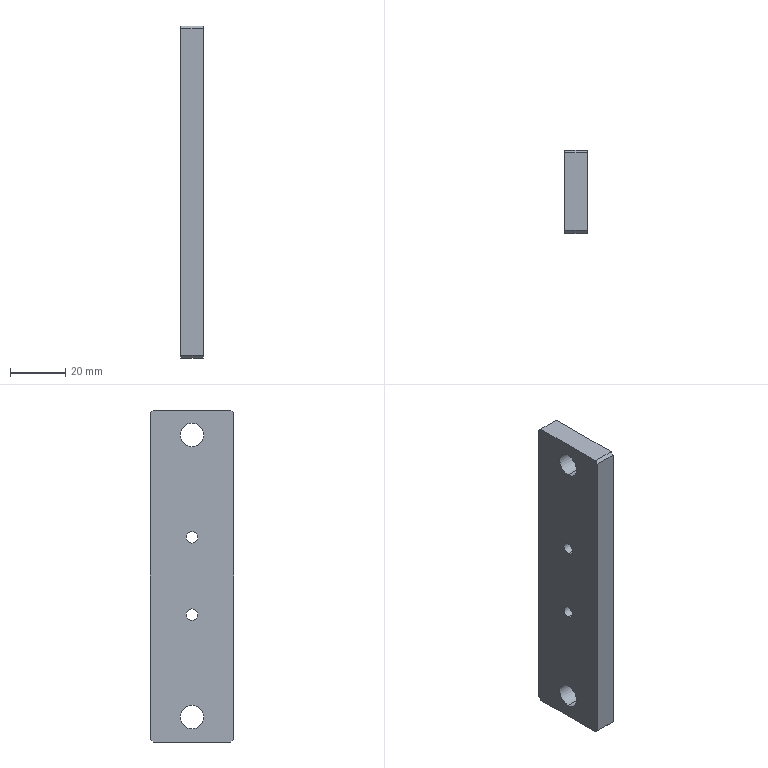Component | SolidWorks | LH-CGJ-01-055-1 | 1 solid | 18 faces | box 8 x 30 x 120 mm | volume 27654 mm3 | plane 10 | cylinder 8 | commonest cylinder face diameters 8.5 x4 4.2 x4 | material A6061
build123d program:
from build123d import *

# Parameters (mm, degrees)
SKETCH1_W                      = 120
SKETCH1_H                      = 30
BOSS_EXTRUDE1_DEPTH            = 8
M5_TAPPED_HOLE1_D              = 4.2
M5_TAPPED_HOLE1_DEPTH          = 12.4
M5_TAPPED_HOLE1_TIP            = 1.262
CHAMFER1_SIZE                  = 1
F_8_5_8_5_DIAMETER_HOLE1_D     = 8.5
F_8_5_8_5_DIAMETER_HOLE1_DEPTH = 12.4
F_8_5_8_5_DIAMETER_HOLE1_TIP   = 2.554


with BuildPart() as part:
    # Sketch1 → Boss-Extrude1 (new body)
    with BuildSketch(Plane.XY):
        with Locations((60, 15)):
            Rectangle(SKETCH1_W, SKETCH1_H)
    extrude(amount=BOSS_EXTRUDE1_DEPTH)

    # M5 Tapped Hole1
    with Locations(Plane.XY.offset(8)):
        with Locations((46, 15), (74, 15)):
            Hole(M5_TAPPED_HOLE1_D / 2, depth=M5_TAPPED_HOLE1_DEPTH)
            with Locations((0, 0, -(M5_TAPPED_HOLE1_DEPTH + M5_TAPPED_HOLE1_TIP / 2))):  # 118° drill point
                Cone(0, M5_TAPPED_HOLE1_D / 2, M5_TAPPED_HOLE1_TIP, mode=Mode.SUBTRACT)

    # Chamfer1
    chamfer1_edges = [part.edges().sort_by_distance(p)[0] for p in [
        (0, 30, 4),
        (120, 30, 4),
        (120, 0, 4),
        (0, 0, 4),
    ]]
    chamfer(chamfer1_edges, length=CHAMFER1_SIZE)

    # 8.5 _8.5_ Diameter Hole1
    with Locations(Plane(origin=(0, 0, 0), x_dir=(-1, 0, 0), z_dir=(0, 0, -1))):
        with Locations((-9, 15), (-111, 15)):
            Hole(F_8_5_8_5_DIAMETER_HOLE1_D / 2, depth=F_8_5_8_5_DIAMETER_HOLE1_DEPTH)
            with Locations((0, 0, -(F_8_5_8_5_DIAMETER_HOLE1_DEPTH + F_8_5_8_5_DIAMETER_HOLE1_TIP / 2))):  # 118° drill point
                Cone(0, F_8_5_8_5_DIAMETER_HOLE1_D / 2, F_8_5_8_5_DIAMETER_HOLE1_TIP, mode=Mode.SUBTRACT)


solid = part.part

# Placed as in the assembly
solid = solid.moved(Location((-38.503, 90.215, 125.05), (0, 90, 0)))
STEP:
#1=COLOUR_RGB('',0.7922,0.8196,0.9333);
#2=FILL_AREA_STYLE_COLOUR('',#1);
#3=FILL_AREA_STYLE('',(#2));
#4=SURFACE_STYLE_FILL_AREA(#3);
#5=SURFACE_SIDE_STYLE('',(#4));
#6=SURFACE_STYLE_USAGE(.BOTH.,#5);
#7=PRESENTATION_STYLE_ASSIGNMENT((#6));
#8=CARTESIAN_POINT('',(-1.516,4.142,0.7205));
#9=VERTEX_POINT('',#8);
#10=CARTESIAN_POINT('',(-1.516,4.142,0.3858));
#11=VERTEX_POINT('',#10);
#12=CARTESIAN_POINT('',(-1.516,4.142,0.5531));
#13=DIRECTION('',(1.,0.,-0.));
#14=DIRECTION('',(0.,0.,-1.));
#15=AXIS2_PLACEMENT_3D('',#12,#13,#14);
#16=CIRCLE('',#15,0.1673);
#17=EDGE_CURVE('',#9,#11,#16,.T.);
#18=ORIENTED_EDGE('',*,*,#17,.F.);
#19=CARTESIAN_POINT('',(-1.201,4.142,0.7205));
#20=VERTEX_POINT('',#19);
#21=CARTESIAN_POINT('',(-1.201,4.142,0.7205));
#22=DIRECTION('',(1.,0.,-0.));
#23=VECTOR('',#22,39.37);
#24=LINE('',#21,#23);
#25=EDGE_CURVE('',#9,#20,#24,.T.);
#26=ORIENTED_EDGE('',*,*,#25,.T.);
#27=CARTESIAN_POINT('',(-1.201,4.142,0.3858));
#28=VERTEX_POINT('',#27);
#29=CARTESIAN_POINT('',(-1.201,4.142,0.5531));
#30=DIRECTION('',(1.,0.,-0.));
#31=DIRECTION('',(-0.,0.,-1.));
#32=AXIS2_PLACEMENT_3D('',#29,#30,#31);
#33=CIRCLE('',#32,0.1673);
#34=EDGE_CURVE('',#20,#28,#33,.T.);
#35=ORIENTED_EDGE('',*,*,#34,.T.);
#36=CARTESIAN_POINT('',(-1.201,4.142,0.3858));
#37=DIRECTION('',(1.,0.,-0.));
#38=VECTOR('',#37,39.37);
#39=LINE('',#36,#38);
#40=EDGE_CURVE('',#11,#28,#39,.T.);
#41=ORIENTED_EDGE('',*,*,#40,.F.);
#42=EDGE_LOOP('',(#18,#26,#35,#41));
#43=FACE_OUTER_BOUND('',#42,.T.);
#44=CARTESIAN_POINT('',(-1.201,4.142,0.5531));
#45=DIRECTION('',(1.,0.,-0.));
#46=DIRECTION('',(-0.,0.,-1.));
#47=AXIS2_PLACEMENT_3D('',#44,#45,#46);
#48=CYLINDRICAL_SURFACE('',#47,0.1673);
#49=ADVANCED_FACE('',(#43),#48,.F.);
#50=CARTESIAN_POINT('',(-1.516,4.142,4.736));
#51=VERTEX_POINT('',#50);
#52=CARTESIAN_POINT('',(-1.516,4.142,4.402));
#53=VERTEX_POINT('',#52);
#54=CARTESIAN_POINT('',(-1.516,4.142,4.569));
#55=DIRECTION('',(1.,0.,-0.));
#56=DIRECTION('',(0.,0.,-1.));
#57=AXIS2_PLACEMENT_3D('',#54,#55,#56);
#58=CIRCLE('',#57,0.1673);
#59=EDGE_CURVE('',#51,#53,#58,.T.);
#60=ORIENTED_EDGE('',*,*,#59,.F.);
#61=CARTESIAN_POINT('',(-1.201,4.142,4.736));
#62=VERTEX_POINT('',#61);
#63=CARTESIAN_POINT('',(-1.201,4.142,4.736));
#64=DIRECTION('',(1.,0.,-0.));
#65=VECTOR('',#64,39.37);
#66=LINE('',#63,#65);
#67=EDGE_CURVE('',#51,#62,#66,.T.);
#68=ORIENTED_EDGE('',*,*,#67,.T.);
#69=CARTESIAN_POINT('',(-1.201,4.142,4.402));
#70=VERTEX_POINT('',#69);
#71=CARTESIAN_POINT('',(-1.201,4.142,4.569));
#72=DIRECTION('',(1.,0.,-0.));
#73=DIRECTION('',(-0.,0.,-1.));
#74=AXIS2_PLACEMENT_3D('',#71,#72,#73);
#75=CIRCLE('',#74,0.1673);
#76=EDGE_CURVE('',#62,#70,#75,.T.);
#77=ORIENTED_EDGE('',*,*,#76,.T.);
#78=CARTESIAN_POINT('',(-1.201,4.142,4.402));
#79=DIRECTION('',(1.,0.,-0.));
#80=VECTOR('',#79,39.37);
#81=LINE('',#78,#80);
#82=EDGE_CURVE('',#53,#70,#81,.T.);
#83=ORIENTED_EDGE('',*,*,#82,.F.);
#84=EDGE_LOOP('',(#60,#68,#77,#83));
#85=FACE_OUTER_BOUND('',#84,.T.);
#86=CARTESIAN_POINT('',(-1.201,4.142,4.569));
#87=DIRECTION('',(1.,0.,-0.));
#88=DIRECTION('',(-0.,0.,-1.));
#89=AXIS2_PLACEMENT_3D('',#86,#87,#88);
#90=CYLINDRICAL_SURFACE('',#89,0.1673);
#91=ADVANCED_FACE('',(#85),#90,.F.);
#92=CARTESIAN_POINT('',(-1.201,4.142,2.093));
#93=VERTEX_POINT('',#92);
#94=CARTESIAN_POINT('',(-1.201,4.142,1.927));
#95=VERTEX_POINT('',#94);
#96=CARTESIAN_POINT('',(-1.201,4.142,2.01));
#97=DIRECTION('',(1.,0.,-0.));
#98=DIRECTION('',(0.,0.,-1.));
#99=AXIS2_PLACEMENT_3D('',#96,#97,#98);
#100=CIRCLE('',#99,0.08268);
#101=EDGE_CURVE('',#93,#95,#100,.T.);
#102=ORIENTED_EDGE('',*,*,#101,.T.);
#103=CARTESIAN_POINT('',(-1.516,4.142,1.927));
#104=VERTEX_POINT('',#103);
#105=CARTESIAN_POINT('',(-1.516,4.142,1.927));
#106=DIRECTION('',(-1.,-0.,0.));
#107=VECTOR('',#106,39.37);
#108=LINE('',#105,#107);
#109=EDGE_CURVE('',#95,#104,#108,.T.);
#110=ORIENTED_EDGE('',*,*,#109,.T.);
#111=CARTESIAN_POINT('',(-1.516,4.142,2.093));
#112=VERTEX_POINT('',#111);
#113=CARTESIAN_POINT('',(-1.516,4.142,2.01));
#114=DIRECTION('',(-1.,-0.,0.));
#115=DIRECTION('',(0.,0.,1.));
#116=AXIS2_PLACEMENT_3D('',#113,#114,#115);
#117=CIRCLE('',#116,0.08268);
#118=EDGE_CURVE('',#104,#112,#117,.T.);
#119=ORIENTED_EDGE('',*,*,#118,.T.);
#120=CARTESIAN_POINT('',(-1.516,4.142,2.093));
#121=DIRECTION('',(-1.,-0.,0.));
#122=VECTOR('',#121,39.37);
#123=LINE('',#120,#122);
#124=EDGE_CURVE('',#93,#112,#123,.T.);
#125=ORIENTED_EDGE('',*,*,#124,.F.);
#126=EDGE_LOOP('',(#102,#110,#119,#125));
#127=FACE_OUTER_BOUND('',#126,.T.);
#128=CARTESIAN_POINT('',(-1.516,4.142,2.01));
#129=DIRECTION('',(-1.,-0.,0.));
#130=DIRECTION('',(0.,0.,1.));
#131=AXIS2_PLACEMENT_3D('',#128,#129,#130);
#132=CYLINDRICAL_SURFACE('',#131,0.08268);
#133=ADVANCED_FACE('',(#127),#132,.F.);
#134=CARTESIAN_POINT('',(-1.201,4.142,3.195));
#135=VERTEX_POINT('',#134);
#136=CARTESIAN_POINT('',(-1.201,4.142,3.03));
#137=VERTEX_POINT('',#136);
#138=CARTESIAN_POINT('',(-1.201,4.142,3.112));
#139=DIRECTION('',(1.,0.,-0.));
#140=DIRECTION('',(0.,0.,-1.));
#141=AXIS2_PLACEMENT_3D('',#138,#139,#140);
#142=CIRCLE('',#141,0.08268);
#143=EDGE_CURVE('',#135,#137,#142,.T.);
#144=ORIENTED_EDGE('',*,*,#143,.T.);
#145=CARTESIAN_POINT('',(-1.516,4.142,3.03));
#146=VERTEX_POINT('',#145);
#147=CARTESIAN_POINT('',(-1.516,4.142,3.03));
#148=DIRECTION('',(-1.,-0.,0.));
#149=VECTOR('',#148,39.37);
#150=LINE('',#147,#149);
#151=EDGE_CURVE('',#137,#146,#150,.T.);
#152=ORIENTED_EDGE('',*,*,#151,.T.);
#153=CARTESIAN_POINT('',(-1.516,4.142,3.195));
#154=VERTEX_POINT('',#153);
#155=CARTESIAN_POINT('',(-1.516,4.142,3.112));
#156=DIRECTION('',(-1.,-0.,0.));
#157=DIRECTION('',(0.,0.,1.));
#158=AXIS2_PLACEMENT_3D('',#155,#156,#157);
#159=CIRCLE('',#158,0.08268);
#160=EDGE_CURVE('',#146,#154,#159,.T.);
#161=ORIENTED_EDGE('',*,*,#160,.T.);
#162=CARTESIAN_POINT('',(-1.516,4.142,3.195));
#163=DIRECTION('',(-1.,-0.,0.));
#164=VECTOR('',#163,39.37);
#165=LINE('',#162,#164);
#166=EDGE_CURVE('',#135,#154,#165,.T.);
#167=ORIENTED_EDGE('',*,*,#166,.F.);
#168=EDGE_LOOP('',(#144,#152,#161,#167));
#169=FACE_OUTER_BOUND('',#168,.T.);
#170=CARTESIAN_POINT('',(-1.516,4.142,3.112));
#171=DIRECTION('',(-1.,-0.,0.));
#172=DIRECTION('',(0.,0.,1.));
#173=AXIS2_PLACEMENT_3D('',#170,#171,#172);
#174=CYLINDRICAL_SURFACE('',#173,0.08268);
#175=ADVANCED_FACE('',(#169),#174,.F.);
#176=CARTESIAN_POINT('',(-1.201,4.694,0.1988));
#177=VERTEX_POINT('',#176);
#178=CARTESIAN_POINT('',(-1.201,3.591,0.1988));
#179=VERTEX_POINT('',#178);
#180=CARTESIAN_POINT('',(-1.201,3.552,0.1988));
#181=DIRECTION('',(0.,-1.,-0.));
#182=VECTOR('',#181,39.37);
#183=LINE('',#180,#182);
#184=EDGE_CURVE('',#177,#179,#183,.T.);
#185=ORIENTED_EDGE('',*,*,#184,.T.);
#186=CARTESIAN_POINT('',(-1.516,3.591,0.1988));
#187=VERTEX_POINT('',#186);
#188=CARTESIAN_POINT('',(-1.516,3.591,0.1988));
#189=DIRECTION('',(-1.,-0.,0.));
#190=VECTOR('',#189,39.37);
#191=LINE('',#188,#190);
#192=EDGE_CURVE('',#179,#187,#191,.T.);
#193=ORIENTED_EDGE('',*,*,#192,.T.);
#194=CARTESIAN_POINT('',(-1.516,4.694,0.1988));
#195=VERTEX_POINT('',#194);
#196=CARTESIAN_POINT('',(-1.516,3.552,0.1988));
#197=DIRECTION('',(0.,-1.,-0.));
#198=VECTOR('',#197,39.37);
#199=LINE('',#196,#198);
#200=EDGE_CURVE('',#195,#187,#199,.T.);
#201=ORIENTED_EDGE('',*,*,#200,.F.);
#202=CARTESIAN_POINT('',(-1.516,4.694,0.1988));
#203=DIRECTION('',(1.,0.,-0.));
#204=VECTOR('',#203,39.37);
#205=LINE('',#202,#204);
#206=EDGE_CURVE('',#195,#177,#205,.T.);
#207=ORIENTED_EDGE('',*,*,#206,.T.);
#208=EDGE_LOOP('',(#185,#193,#201,#207));
#209=FACE_OUTER_BOUND('',#208,.T.);
#210=CARTESIAN_POINT('',(-1.516,3.552,0.1988));
#211=DIRECTION('',(0.,-0.,1.));
#212=DIRECTION('',(1.,0.,-0.));
#213=AXIS2_PLACEMENT_3D('',#210,#211,#212);
#214=PLANE('',#213);
#215=ADVANCED_FACE('',(#209),#214,.F.);
#216=CARTESIAN_POINT('',(-1.516,3.552,0.2382));
#217=VERTEX_POINT('',#216);
#218=CARTESIAN_POINT('',(-1.516,3.552,4.884));
#219=VERTEX_POINT('',#218);
#220=CARTESIAN_POINT('',(-1.516,3.552,0.1988));
#221=DIRECTION('',(0.,-0.,1.));
#222=VECTOR('',#221,39.37);
#223=LINE('',#220,#222);
#224=EDGE_CURVE('',#217,#219,#223,.T.);
#225=ORIENTED_EDGE('',*,*,#224,.F.);
#226=CARTESIAN_POINT('',(-1.201,3.552,0.2382));
#227=VERTEX_POINT('',#226);
#228=CARTESIAN_POINT('',(-1.516,3.552,0.2382));
#229=DIRECTION('',(1.,0.,-0.));
#230=VECTOR('',#229,39.37);
#231=LINE('',#228,#230);
#232=EDGE_CURVE('',#217,#227,#231,.T.);
#233=ORIENTED_EDGE('',*,*,#232,.T.);
#234=CARTESIAN_POINT('',(-1.201,3.552,4.884));
#235=VERTEX_POINT('',#234);
#236=CARTESIAN_POINT('',(-1.201,3.552,0.1988));
#237=DIRECTION('',(0.,-0.,1.));
#238=VECTOR('',#237,39.37);
#239=LINE('',#236,#238);
#240=EDGE_CURVE('',#227,#235,#239,.T.);
#241=ORIENTED_EDGE('',*,*,#240,.T.);
#242=CARTESIAN_POINT('',(-1.516,3.552,4.884));
#243=DIRECTION('',(-1.,-0.,0.));
#244=VECTOR('',#243,39.37);
#245=LINE('',#242,#244);
#246=EDGE_CURVE('',#235,#219,#245,.T.);
#247=ORIENTED_EDGE('',*,*,#246,.T.);
#248=EDGE_LOOP('',(#225,#233,#241,#247));
#249=FACE_OUTER_BOUND('',#248,.T.);
#250=CARTESIAN_POINT('',(-1.516,3.552,0.1988));
#251=DIRECTION('',(-0.,1.,0.));
#252=DIRECTION('',(-1.,-0.,0.));
#253=AXIS2_PLACEMENT_3D('',#250,#251,#252);
#254=PLANE('',#253);
#255=ADVANCED_FACE('',(#249),#254,.F.);
#256=CARTESIAN_POINT('',(-1.516,3.591,4.923));
#257=VERTEX_POINT('',#256);
#258=CARTESIAN_POINT('',(-1.516,4.694,4.923));
#259=VERTEX_POINT('',#258);
#260=CARTESIAN_POINT('',(-1.516,3.552,4.923));
#261=DIRECTION('',(-0.,1.,0.));
#262=VECTOR('',#261,39.37);
#263=LINE('',#260,#262);
#264=EDGE_CURVE('',#257,#259,#263,.T.);
#265=ORIENTED_EDGE('',*,*,#264,.F.);
#266=CARTESIAN_POINT('',(-1.201,3.591,4.923));
#267=VERTEX_POINT('',#266);
#268=CARTESIAN_POINT('',(-1.516,3.591,4.923));
#269=DIRECTION('',(1.,0.,-0.));
#270=VECTOR('',#269,39.37);
#271=LINE('',#268,#270);
#272=EDGE_CURVE('',#257,#267,#271,.T.);
#273=ORIENTED_EDGE('',*,*,#272,.T.);
#274=CARTESIAN_POINT('',(-1.201,4.694,4.923));
#275=VERTEX_POINT('',#274);
#276=CARTESIAN_POINT('',(-1.201,3.552,4.923));
#277=DIRECTION('',(-0.,1.,0.));
#278=VECTOR('',#277,39.37);
#279=LINE('',#276,#278);
#280=EDGE_CURVE('',#267,#275,#279,.T.);
#281=ORIENTED_EDGE('',*,*,#280,.T.);
#282=CARTESIAN_POINT('',(-1.516,4.694,4.923));
#283=DIRECTION('',(-1.,-0.,0.));
#284=VECTOR('',#283,39.37);
#285=LINE('',#282,#284);
#286=EDGE_CURVE('',#275,#259,#285,.T.);
#287=ORIENTED_EDGE('',*,*,#286,.T.);
#288=EDGE_LOOP('',(#265,#273,#281,#287));
#289=FACE_OUTER_BOUND('',#288,.T.);
#290=CARTESIAN_POINT('',(-1.516,3.552,4.923));
#291=DIRECTION('',(-0.,0.,-1.));
#292=DIRECTION('',(-1.,-0.,0.));
#293=AXIS2_PLACEMENT_3D('',#290,#291,#292);
#294=PLANE('',#293);
#295=ADVANCED_FACE('',(#289),#294,.F.);
#296=CARTESIAN_POINT('',(-1.201,4.733,4.884));
#297=VERTEX_POINT('',#296);
#298=CARTESIAN_POINT('',(-1.201,4.733,0.2382));
#299=VERTEX_POINT('',#298);
#300=CARTESIAN_POINT('',(-1.201,4.733,0.1988));
#301=DIRECTION('',(-0.,0.,-1.));
#302=VECTOR('',#301,39.37);
#303=LINE('',#300,#302);
#304=EDGE_CURVE('',#297,#299,#303,.T.);
#305=ORIENTED_EDGE('',*,*,#304,.T.);
#306=CARTESIAN_POINT('',(-1.516,4.733,0.2382));
#307=VERTEX_POINT('',#306);
#308=CARTESIAN_POINT('',(-1.516,4.733,0.2382));
#309=DIRECTION('',(-1.,-0.,0.));
#310=VECTOR('',#309,39.37);
#311=LINE('',#308,#310);
#312=EDGE_CURVE('',#299,#307,#311,.T.);
#313=ORIENTED_EDGE('',*,*,#312,.T.);
#314=CARTESIAN_POINT('',(-1.516,4.733,4.884));
#315=VERTEX_POINT('',#314);
#316=CARTESIAN_POINT('',(-1.516,4.733,0.1988));
#317=DIRECTION('',(-0.,0.,-1.));
#318=VECTOR('',#317,39.37);
#319=LINE('',#316,#318);
#320=EDGE_CURVE('',#315,#307,#319,.T.);
#321=ORIENTED_EDGE('',*,*,#320,.F.);
#322=CARTESIAN_POINT('',(-1.516,4.733,4.884));
#323=DIRECTION('',(1.,0.,-0.));
#324=VECTOR('',#323,39.37);
#325=LINE('',#322,#324);
#326=EDGE_CURVE('',#315,#297,#325,.T.);
#327=ORIENTED_EDGE('',*,*,#326,.T.);
#328=EDGE_LOOP('',(#305,#313,#321,#327));
#329=FACE_OUTER_BOUND('',#328,.T.);
#330=CARTESIAN_POINT('',(-1.516,4.733,0.1988));
#331=DIRECTION('',(0.,-1.,-0.));
#332=DIRECTION('',(1.,0.,-0.));
#333=AXIS2_PLACEMENT_3D('',#330,#331,#332);
#334=PLANE('',#333);
#335=ADVANCED_FACE('',(#329),#334,.F.);
#336=CARTESIAN_POINT('',(-1.516,4.142,0.5531));
#337=DIRECTION('',(1.,0.,-0.));
#338=DIRECTION('',(0.,0.,-1.));
#339=AXIS2_PLACEMENT_3D('',#336,#337,#338);
#340=CIRCLE('',#339,0.1673);
#341=EDGE_CURVE('',#11,#9,#340,.T.);
#342=ORIENTED_EDGE('',*,*,#341,.T.);
#343=ORIENTED_EDGE('',*,*,#17,.T.);
#344=EDGE_LOOP('',(#342,#343));
#345=FACE_BOUND('',#344,.T.);
#346=CARTESIAN_POINT('',(-1.516,4.142,4.569));
#347=DIRECTION('',(1.,0.,-0.));
#348=DIRECTION('',(0.,0.,-1.));
#349=AXIS2_PLACEMENT_3D('',#346,#347,#348);
#350=CIRCLE('',#349,0.1673);
#351=EDGE_CURVE('',#53,#51,#350,.T.);
#352=ORIENTED_EDGE('',*,*,#351,.T.);
#353=ORIENTED_EDGE('',*,*,#59,.T.);
#354=EDGE_LOOP('',(#352,#353));
#355=FACE_BOUND('',#354,.T.);
#356=CARTESIAN_POINT('',(-1.516,4.142,2.01));
#357=DIRECTION('',(-1.,-0.,0.));
#358=DIRECTION('',(0.,0.,1.));
#359=AXIS2_PLACEMENT_3D('',#356,#357,#358);
#360=CIRCLE('',#359,0.08268);
#361=EDGE_CURVE('',#112,#104,#360,.T.);
#362=ORIENTED_EDGE('',*,*,#361,.F.);
#363=ORIENTED_EDGE('',*,*,#118,.F.);
#364=EDGE_LOOP('',(#362,#363));
#365=FACE_BOUND('',#364,.T.);
#366=CARTESIAN_POINT('',(-1.516,4.142,3.112));
#367=DIRECTION('',(-1.,-0.,0.));
#368=DIRECTION('',(0.,0.,1.));
#369=AXIS2_PLACEMENT_3D('',#366,#367,#368);
#370=CIRCLE('',#369,0.08268);
#371=EDGE_CURVE('',#154,#146,#370,.T.);
#372=ORIENTED_EDGE('',*,*,#371,.F.);
#373=ORIENTED_EDGE('',*,*,#160,.F.);
#374=EDGE_LOOP('',(#372,#373));
#375=FACE_BOUND('',#374,.T.);
#376=ORIENTED_EDGE('',*,*,#200,.T.);
#377=CARTESIAN_POINT('',(-1.516,3.552,0.2382));
#378=DIRECTION('',(0.,-0.7071,0.7071));
#379=VECTOR('',#378,39.37);
#380=LINE('',#377,#379);
#381=EDGE_CURVE('',#187,#217,#380,.T.);
#382=ORIENTED_EDGE('',*,*,#381,.T.);
#383=ORIENTED_EDGE('',*,*,#224,.T.);
#384=CARTESIAN_POINT('',(-1.516,3.591,4.923));
#385=DIRECTION('',(0.,0.7071,0.7071));
#386=VECTOR('',#385,39.37);
#387=LINE('',#384,#386);
#388=EDGE_CURVE('',#219,#257,#387,.T.);
#389=ORIENTED_EDGE('',*,*,#388,.T.);
#390=ORIENTED_EDGE('',*,*,#264,.T.);
#391=CARTESIAN_POINT('',(-1.516,4.733,4.884));
#392=DIRECTION('',(-0.,0.7071,-0.7071));
#393=VECTOR('',#392,39.37);
#394=LINE('',#391,#393);
#395=EDGE_CURVE('',#259,#315,#394,.T.);
#396=ORIENTED_EDGE('',*,*,#395,.T.);
#397=ORIENTED_EDGE('',*,*,#320,.T.);
#398=CARTESIAN_POINT('',(-1.516,4.694,0.1988));
#399=DIRECTION('',(-0.,-0.7071,-0.7071));
#400=VECTOR('',#399,39.37);
#401=LINE('',#398,#400);
#402=EDGE_CURVE('',#307,#195,#401,.T.);
#403=ORIENTED_EDGE('',*,*,#402,.T.);
#404=EDGE_LOOP('',(#376,#382,#383,#389,#390,#396,#397,#403));
#405=FACE_OUTER_BOUND('',#404,.T.);
#406=CARTESIAN_POINT('',(-1.516,3.552,0.1988));
#407=DIRECTION('',(1.,0.,-0.));
#408=DIRECTION('',(-0.,0.,-1.));
#409=AXIS2_PLACEMENT_3D('',#406,#407,#408);
#410=PLANE('',#409);
#411=ADVANCED_FACE('',(#345,#355,#365,#375,#405),#410,.F.);
#412=CARTESIAN_POINT('',(-1.201,4.142,0.5531));
#413=DIRECTION('',(1.,0.,-0.));
#414=DIRECTION('',(-0.,0.,-1.));
#415=AXIS2_PLACEMENT_3D('',#412,#413,#414);
#416=CIRCLE('',#415,0.1673);
#417=EDGE_CURVE('',#28,#20,#416,.T.);
#418=ORIENTED_EDGE('',*,*,#417,.F.);
#419=ORIENTED_EDGE('',*,*,#34,.F.);
#420=EDGE_LOOP('',(#418,#419));
#421=FACE_BOUND('',#420,.T.);
#422=CARTESIAN_POINT('',(-1.201,4.142,4.569));
#423=DIRECTION('',(1.,0.,-0.));
#424=DIRECTION('',(-0.,0.,-1.));
#425=AXIS2_PLACEMENT_3D('',#422,#423,#424);
#426=CIRCLE('',#425,0.1673);
#427=EDGE_CURVE('',#70,#62,#426,.T.);
#428=ORIENTED_EDGE('',*,*,#427,.F.);
#429=ORIENTED_EDGE('',*,*,#76,.F.);
#430=EDGE_LOOP('',(#428,#429));
#431=FACE_BOUND('',#430,.T.);
#432=ORIENTED_EDGE('',*,*,#101,.F.);
#433=CARTESIAN_POINT('',(-1.201,4.142,2.01));
#434=DIRECTION('',(1.,0.,-0.));
#435=DIRECTION('',(0.,0.,-1.));
#436=AXIS2_PLACEMENT_3D('',#433,#434,#435);
#437=CIRCLE('',#436,0.08268);
#438=EDGE_CURVE('',#95,#93,#437,.T.);
#439=ORIENTED_EDGE('',*,*,#438,.F.);
#440=EDGE_LOOP('',(#432,#439));
#441=FACE_BOUND('',#440,.T.);
#442=ORIENTED_EDGE('',*,*,#143,.F.);
#443=CARTESIAN_POINT('',(-1.201,4.142,3.112));
#444=DIRECTION('',(1.,0.,-0.));
#445=DIRECTION('',(0.,0.,-1.));
#446=AXIS2_PLACEMENT_3D('',#443,#444,#445);
#447=CIRCLE('',#446,0.08268);
#448=EDGE_CURVE('',#137,#135,#447,.T.);
#449=ORIENTED_EDGE('',*,*,#448,.F.);
#450=EDGE_LOOP('',(#442,#449));
#451=FACE_BOUND('',#450,.T.);
#452=ORIENTED_EDGE('',*,*,#240,.F.);
#453=CARTESIAN_POINT('',(-1.201,3.571,0.2185));
#454=DIRECTION('',(-0.,0.7071,-0.7071));
#455=VECTOR('',#454,39.37);
#456=LINE('',#453,#455);
#457=EDGE_CURVE('',#227,#179,#456,.T.);
#458=ORIENTED_EDGE('',*,*,#457,.T.);
#459=ORIENTED_EDGE('',*,*,#184,.F.);
#460=CARTESIAN_POINT('',(-1.201,4.123,-0.372));
#461=DIRECTION('',(0.,0.7071,0.7071));
#462=VECTOR('',#461,39.37);
#463=LINE('',#460,#462);
#464=EDGE_CURVE('',#177,#299,#463,.T.);
#465=ORIENTED_EDGE('',*,*,#464,.T.);
#466=ORIENTED_EDGE('',*,*,#304,.F.);
#467=CARTESIAN_POINT('',(-1.201,6.485,3.132));
#468=DIRECTION('',(0.,-0.7071,0.7071));
#469=VECTOR('',#468,39.37);
#470=LINE('',#467,#469);
#471=EDGE_CURVE('',#297,#275,#470,.T.);
#472=ORIENTED_EDGE('',*,*,#471,.T.);
#473=ORIENTED_EDGE('',*,*,#280,.F.);
#474=CARTESIAN_POINT('',(-1.201,1.209,2.541));
#475=DIRECTION('',(-0.,-0.7071,-0.7071));
#476=VECTOR('',#475,39.37);
#477=LINE('',#474,#476);
#478=EDGE_CURVE('',#267,#235,#477,.T.);
#479=ORIENTED_EDGE('',*,*,#478,.T.);
#480=EDGE_LOOP('',(#452,#458,#459,#465,#466,#472,#473,#479));
#481=FACE_OUTER_BOUND('',#480,.T.);
#482=CARTESIAN_POINT('',(-1.201,3.552,0.1988));
#483=DIRECTION('',(1.,0.,-0.));
#484=DIRECTION('',(-0.,0.,-1.));
#485=AXIS2_PLACEMENT_3D('',#482,#483,#484);
#486=PLANE('',#485);
#487=ADVANCED_FACE('',(#421,#431,#441,#451,#481),#486,.T.);
#488=ORIENTED_EDGE('',*,*,#151,.F.);
#489=ORIENTED_EDGE('',*,*,#448,.T.);
#490=ORIENTED_EDGE('',*,*,#166,.T.);
#491=ORIENTED_EDGE('',*,*,#371,.T.);
#492=EDGE_LOOP('',(#488,#489,#490,#491));
#493=FACE_OUTER_BOUND('',#492,.T.);
#494=CARTESIAN_POINT('',(-1.516,4.142,3.112));
#495=DIRECTION('',(-1.,-0.,0.));
#496=DIRECTION('',(0.,0.,1.));
#497=AXIS2_PLACEMENT_3D('',#494,#495,#496);
#498=CYLINDRICAL_SURFACE('',#497,0.08268);
#499=ADVANCED_FACE('',(#493),#498,.F.);
#500=ORIENTED_EDGE('',*,*,#109,.F.);
#501=ORIENTED_EDGE('',*,*,#438,.T.);
#502=ORIENTED_EDGE('',*,*,#124,.T.);
#503=ORIENTED_EDGE('',*,*,#361,.T.);
#504=EDGE_LOOP('',(#500,#501,#502,#503));
#505=FACE_OUTER_BOUND('',#504,.T.);
#506=CARTESIAN_POINT('',(-1.516,4.142,2.01));
#507=DIRECTION('',(-1.,-0.,0.));
#508=DIRECTION('',(0.,0.,1.));
#509=AXIS2_PLACEMENT_3D('',#506,#507,#508);
#510=CYLINDRICAL_SURFACE('',#509,0.08268);
#511=ADVANCED_FACE('',(#505),#510,.F.);
#512=ORIENTED_EDGE('',*,*,#381,.F.);
#513=ORIENTED_EDGE('',*,*,#192,.F.);
#514=ORIENTED_EDGE('',*,*,#457,.F.);
#515=ORIENTED_EDGE('',*,*,#232,.F.);
#516=EDGE_LOOP('',(#512,#513,#514,#515));
#517=FACE_OUTER_BOUND('',#516,.T.);
#518=CARTESIAN_POINT('',(-1.516,3.552,0.2382));
#519=DIRECTION('',(0.,0.7071,0.7071));
#520=DIRECTION('',(1.,0.,-0.));
#521=AXIS2_PLACEMENT_3D('',#518,#519,#520);
#522=PLANE('',#521);
#523=ADVANCED_FACE('',(#517),#522,.F.);
#524=ORIENTED_EDGE('',*,*,#402,.F.);
#525=ORIENTED_EDGE('',*,*,#312,.F.);
#526=ORIENTED_EDGE('',*,*,#464,.F.);
#527=ORIENTED_EDGE('',*,*,#206,.F.);
#528=EDGE_LOOP('',(#524,#525,#526,#527));
#529=FACE_OUTER_BOUND('',#528,.T.);
#530=CARTESIAN_POINT('',(-1.516,4.694,0.1988));
#531=DIRECTION('',(0.,-0.7071,0.7071));
#532=DIRECTION('',(1.,0.,-0.));
#533=AXIS2_PLACEMENT_3D('',#530,#531,#532);
#534=PLANE('',#533);
#535=ADVANCED_FACE('',(#529),#534,.F.);
#536=ORIENTED_EDGE('',*,*,#388,.F.);
#537=ORIENTED_EDGE('',*,*,#246,.F.);
#538=ORIENTED_EDGE('',*,*,#478,.F.);
#539=ORIENTED_EDGE('',*,*,#272,.F.);
#540=EDGE_LOOP('',(#536,#537,#538,#539));
#541=FACE_OUTER_BOUND('',#540,.T.);
#542=CARTESIAN_POINT('',(-1.516,3.591,4.923));
#543=DIRECTION('',(-0.,0.7071,-0.7071));
#544=DIRECTION('',(1.,0.,-0.));
#545=AXIS2_PLACEMENT_3D('',#542,#543,#544);
#546=PLANE('',#545);
#547=ADVANCED_FACE('',(#541),#546,.F.);
#548=ORIENTED_EDGE('',*,*,#395,.F.);
#549=ORIENTED_EDGE('',*,*,#286,.F.);
#550=ORIENTED_EDGE('',*,*,#471,.F.);
#551=ORIENTED_EDGE('',*,*,#326,.F.);
#552=EDGE_LOOP('',(#548,#549,#550,#551));
#553=FACE_OUTER_BOUND('',#552,.T.);
#554=CARTESIAN_POINT('',(-1.516,4.733,4.884));
#555=DIRECTION('',(-0.,-0.7071,-0.7071));
#556=DIRECTION('',(1.,0.,-0.));
#557=AXIS2_PLACEMENT_3D('',#554,#555,#556);
#558=PLANE('',#557);
#559=ADVANCED_FACE('',(#553),#558,.F.);
#560=ORIENTED_EDGE('',*,*,#67,.F.);
#561=ORIENTED_EDGE('',*,*,#351,.F.);
#562=ORIENTED_EDGE('',*,*,#82,.T.);
#563=ORIENTED_EDGE('',*,*,#427,.T.);
#564=EDGE_LOOP('',(#560,#561,#562,#563));
#565=FACE_OUTER_BOUND('',#564,.T.);
#566=CARTESIAN_POINT('',(-1.201,4.142,4.569));
#567=DIRECTION('',(1.,0.,-0.));
#568=DIRECTION('',(-0.,0.,-1.));
#569=AXIS2_PLACEMENT_3D('',#566,#567,#568);
#570=CYLINDRICAL_SURFACE('',#569,0.1673);
#571=ADVANCED_FACE('',(#565),#570,.F.);
#572=ORIENTED_EDGE('',*,*,#25,.F.);
#573=ORIENTED_EDGE('',*,*,#341,.F.);
#574=ORIENTED_EDGE('',*,*,#40,.T.);
#575=ORIENTED_EDGE('',*,*,#417,.T.);
#576=EDGE_LOOP('',(#572,#573,#574,#575));
#577=FACE_OUTER_BOUND('',#576,.T.);
#578=CARTESIAN_POINT('',(-1.201,4.142,0.5531));
#579=DIRECTION('',(1.,0.,-0.));
#580=DIRECTION('',(-0.,0.,-1.));
#581=AXIS2_PLACEMENT_3D('',#578,#579,#580);
#582=CYLINDRICAL_SURFACE('',#581,0.1673);
#583=ADVANCED_FACE('',(#577),#582,.F.);
#584=CLOSED_SHELL('',(#49,#91,#133,#175,#215,#255,#295,#335,#411,#487,#499,#511,#523,#535,#547,#559,#571,#583));
#585=MANIFOLD_SOLID_BREP('',#584);
#586=STYLED_ITEM('',(#7),#585);
#587=(LENGTH_UNIT()NAMED_UNIT(*)SI_UNIT($,.METRE.));
#588=LENGTH_MEASURE_WITH_UNIT(LENGTH_MEASURE(0.0254),#587);
#589=DIMENSIONAL_EXPONENTS(1.,0.,0.,0.,0.,0.,0.);
#590=(CONVERSION_BASED_UNIT('',#588)LENGTH_UNIT()NAMED_UNIT(#589));
#591=UNCERTAINTY_MEASURE_WITH_UNIT(LENGTH_MEASURE(0.00001),#590,'','');
#592=(NAMED_UNIT(*)PLANE_ANGLE_UNIT()SI_UNIT($,.RADIAN.));
#593=(NAMED_UNIT(*)SI_UNIT($,.STERADIAN.)SOLID_ANGLE_UNIT());
#594=(GEOMETRIC_REPRESENTATION_CONTEXT(3)GLOBAL_UNCERTAINTY_ASSIGNED_CONTEXT((#591))GLOBAL_UNIT_ASSIGNED_CONTEXT((#590,#592,#593))REPRESENTATION_CONTEXT('',''));
#595=MECHANICAL_DESIGN_GEOMETRIC_PRESENTATION_REPRESENTATION('',(#586),#594);
#596=CARTESIAN_POINT('',(0.,0.,0.));
#597=DIRECTION('',(0.,0.,1.));
#598=DIRECTION('',(1.,0.,0.));
#599=AXIS2_PLACEMENT_3D('',#596,#597,#598);
#600=(LENGTH_UNIT()NAMED_UNIT(*)SI_UNIT($,.METRE.));
#601=LENGTH_MEASURE_WITH_UNIT(LENGTH_MEASURE(0.0254),#600);
#602=DIMENSIONAL_EXPONENTS(1.,0.,0.,0.,0.,0.,0.);
#603=(CONVERSION_BASED_UNIT('',#601)LENGTH_UNIT()NAMED_UNIT(#602));
#604=UNCERTAINTY_MEASURE_WITH_UNIT(LENGTH_MEASURE(0.00001),#603,'','');
#605=(NAMED_UNIT(*)PLANE_ANGLE_UNIT()SI_UNIT($,.RADIAN.));
#606=(NAMED_UNIT(*)SI_UNIT($,.STERADIAN.)SOLID_ANGLE_UNIT());
#607=(GEOMETRIC_REPRESENTATION_CONTEXT(3)GLOBAL_UNCERTAINTY_ASSIGNED_CONTEXT((#604))GLOBAL_UNIT_ASSIGNED_CONTEXT((#603,#605,#606))REPRESENTATION_CONTEXT('',''));
#608=ADVANCED_BREP_SHAPE_REPRESENTATION('',(#585,#599),#607);
#609=PRESENTATION_LAYER_ASSIGNMENT('','',(#586));